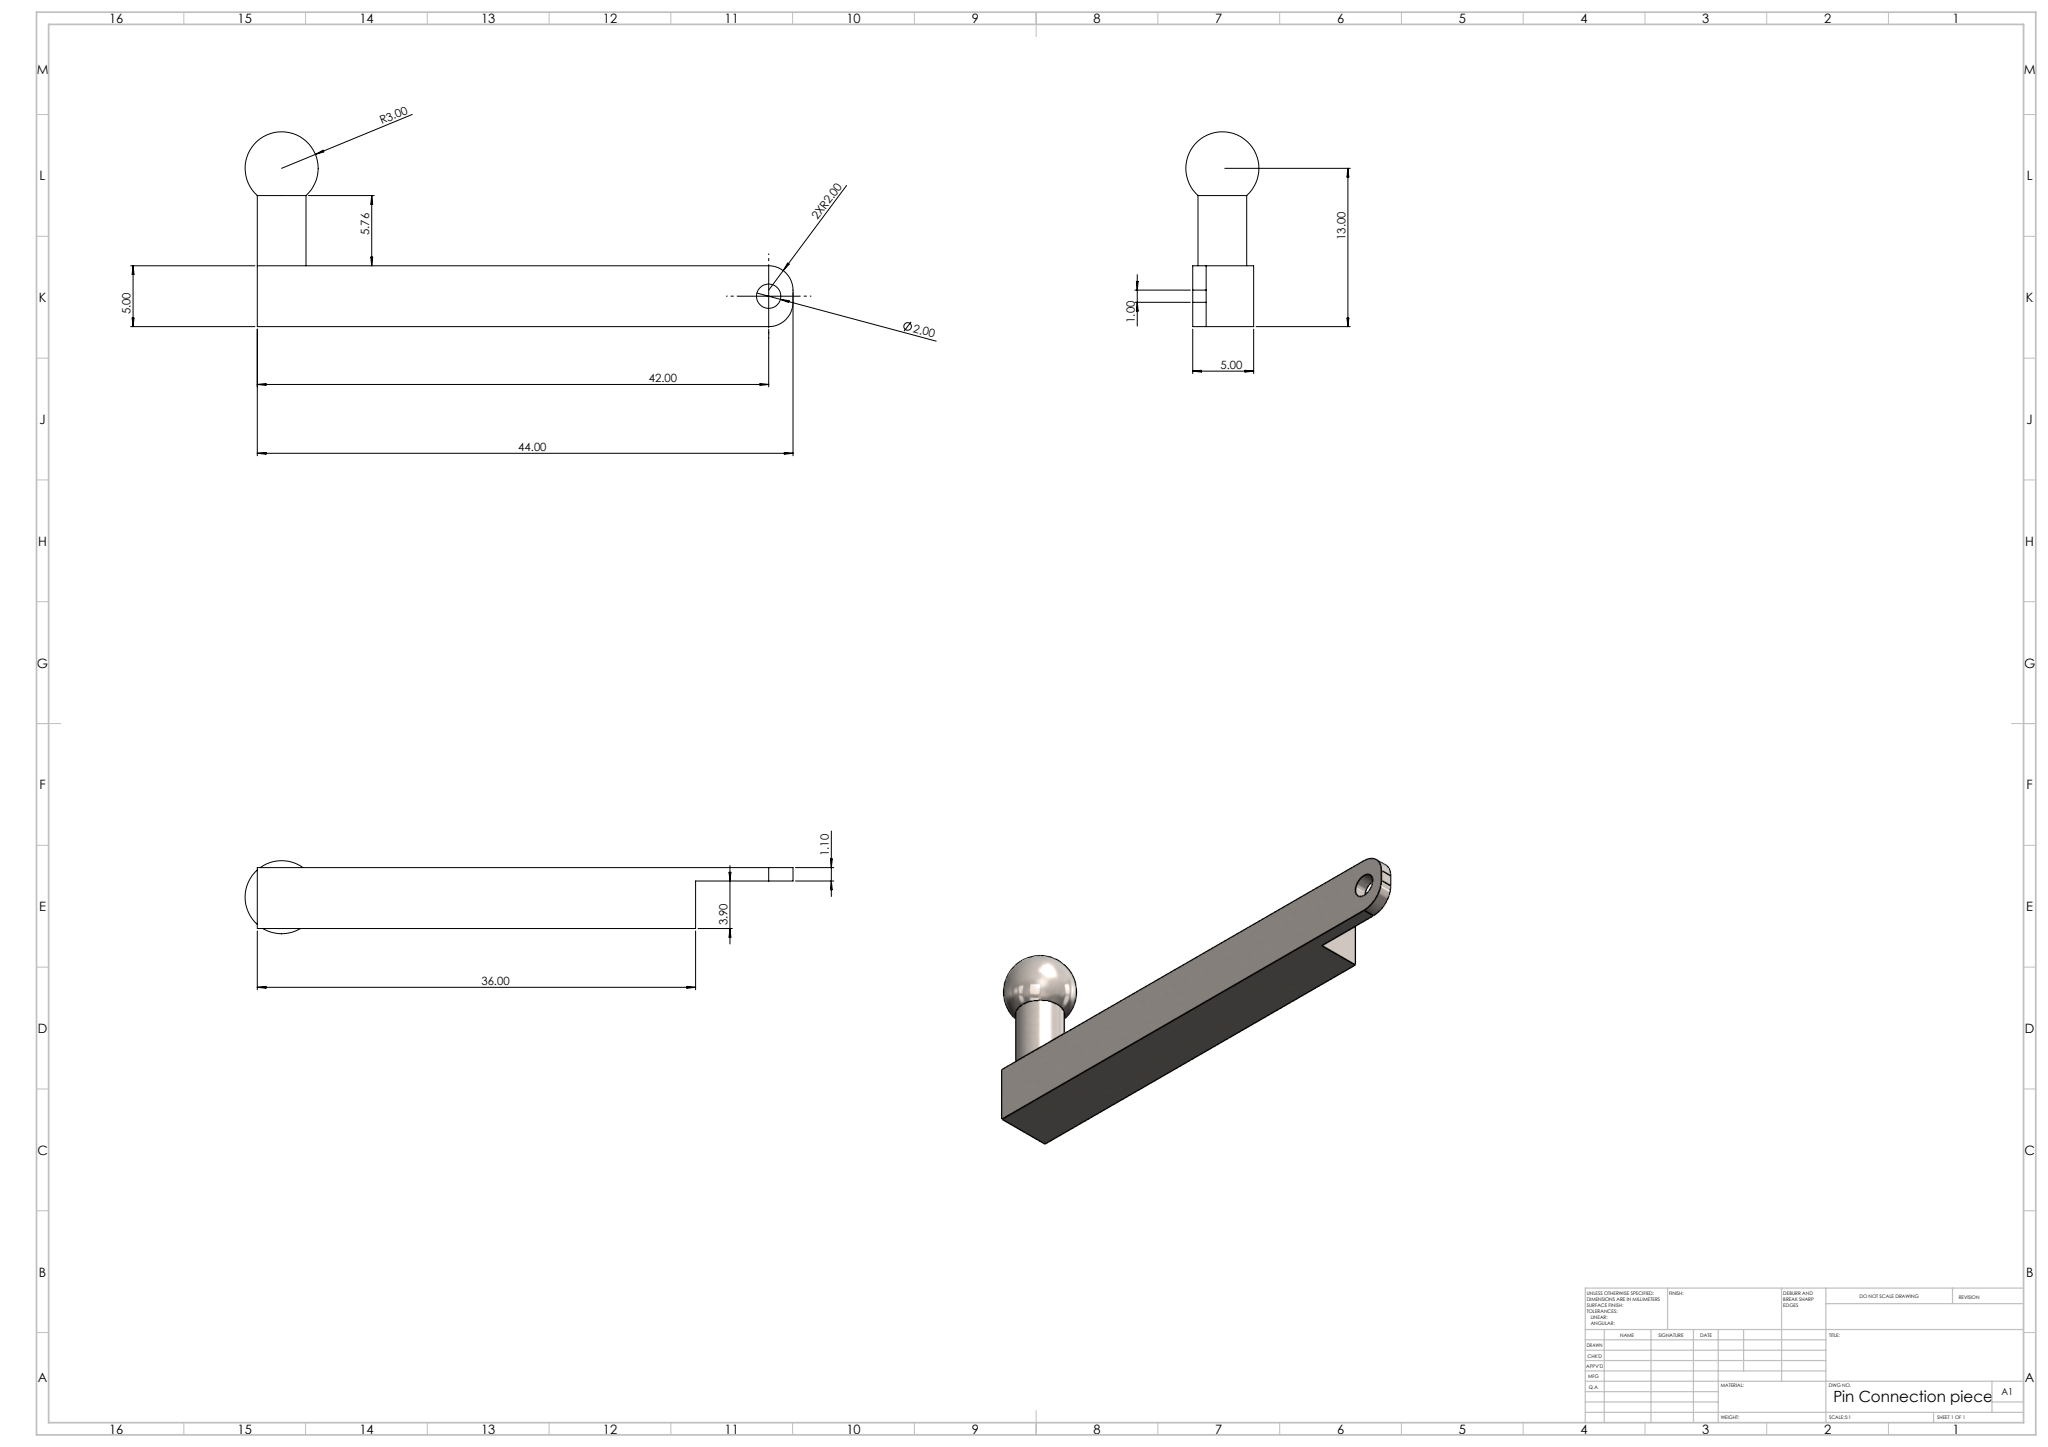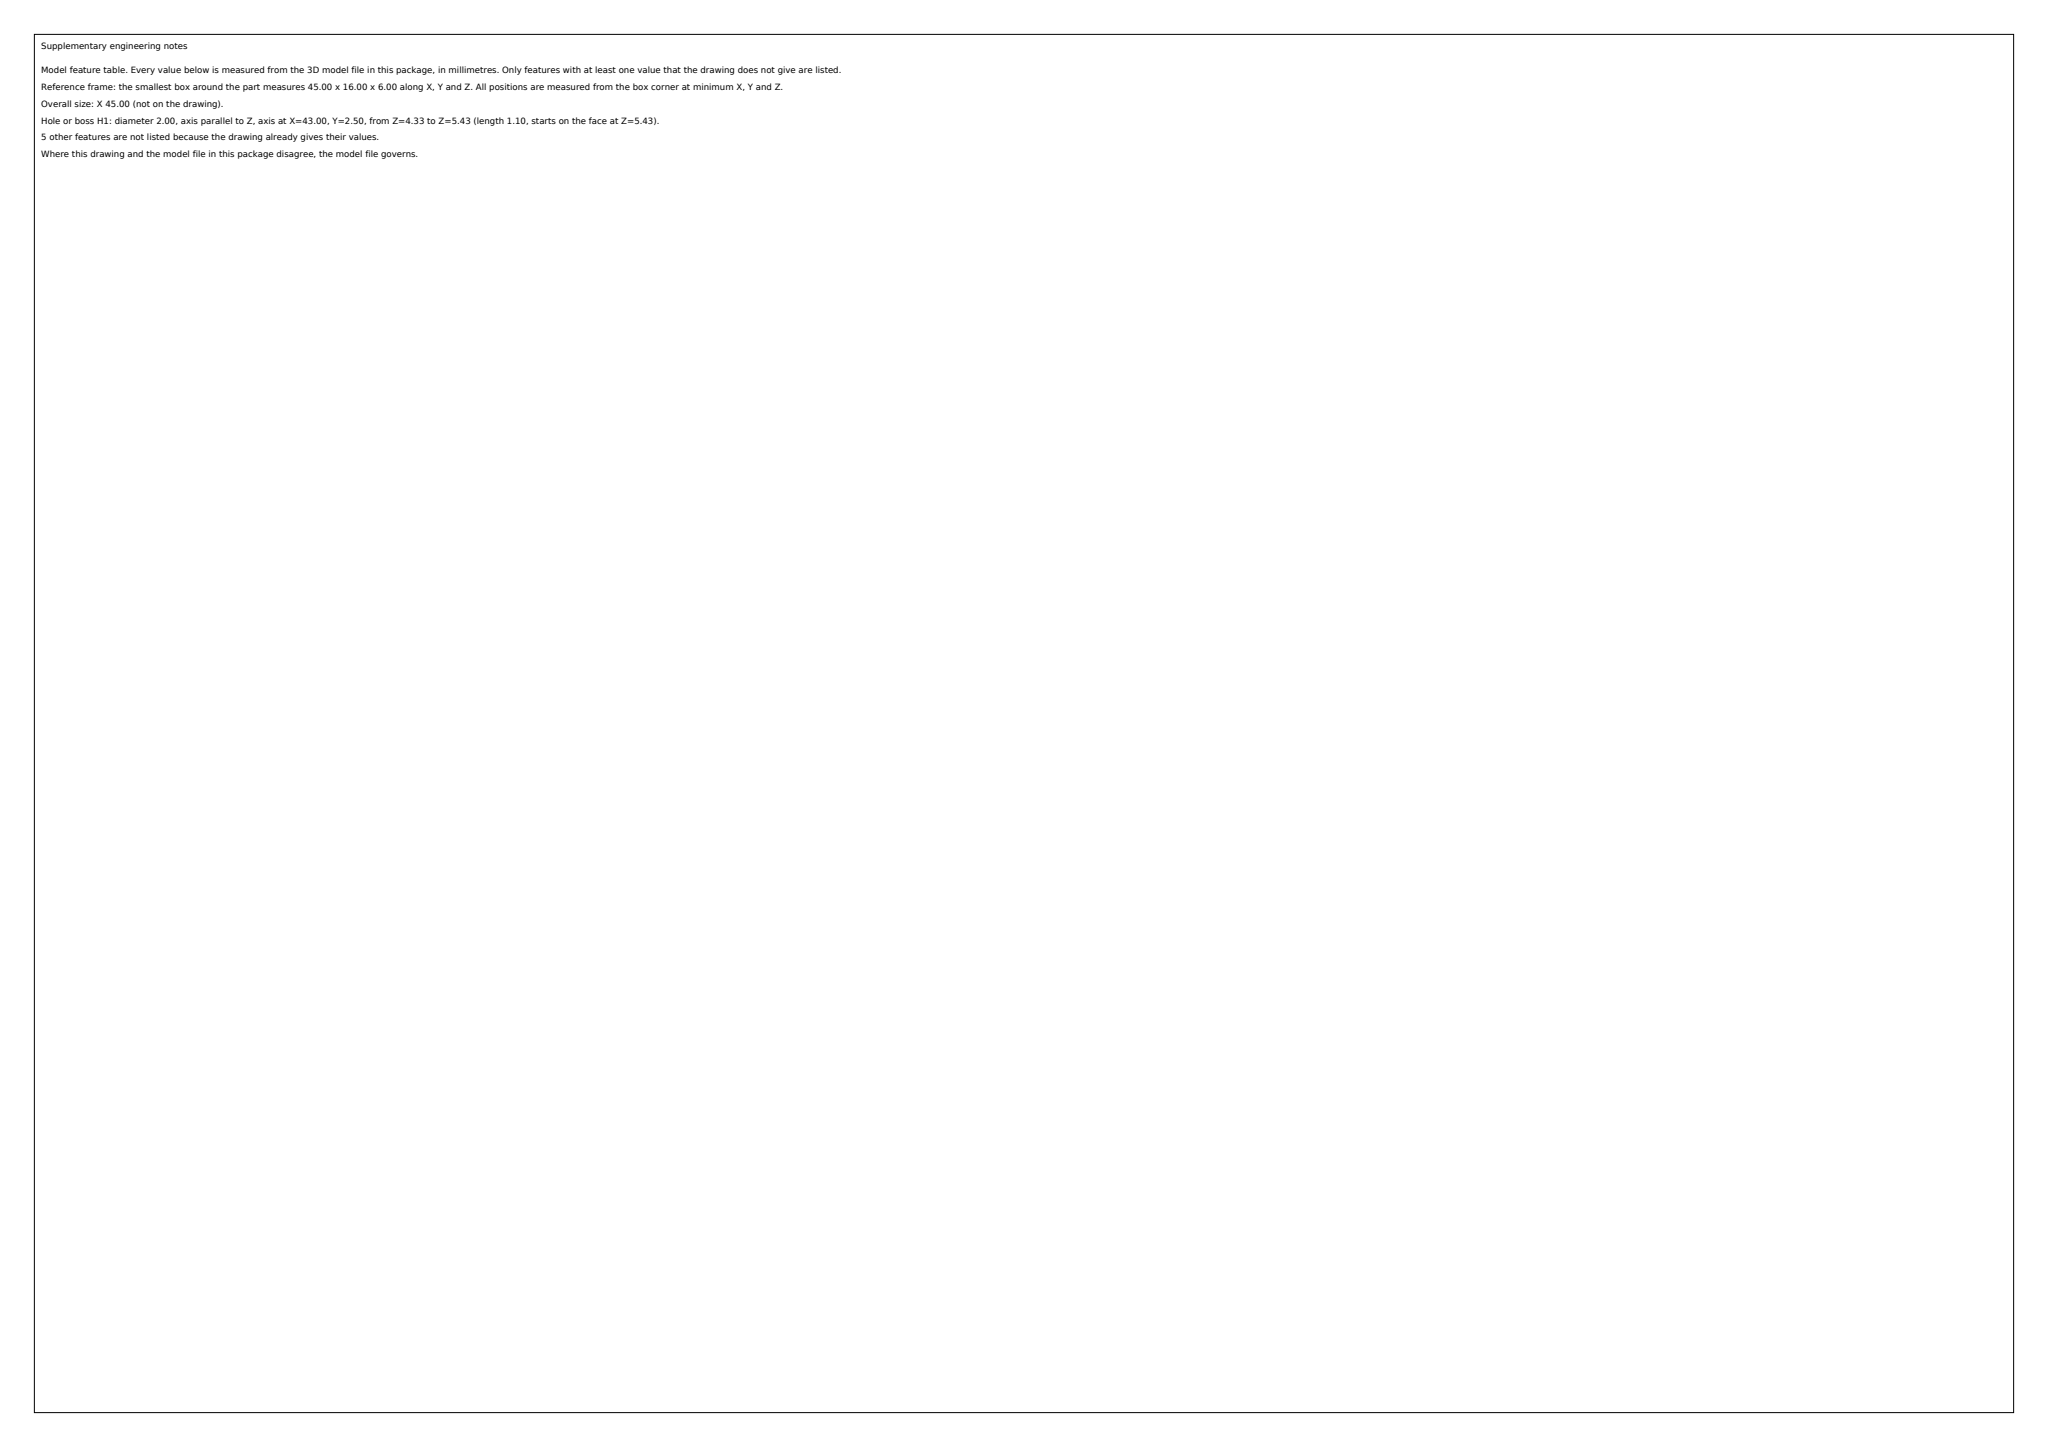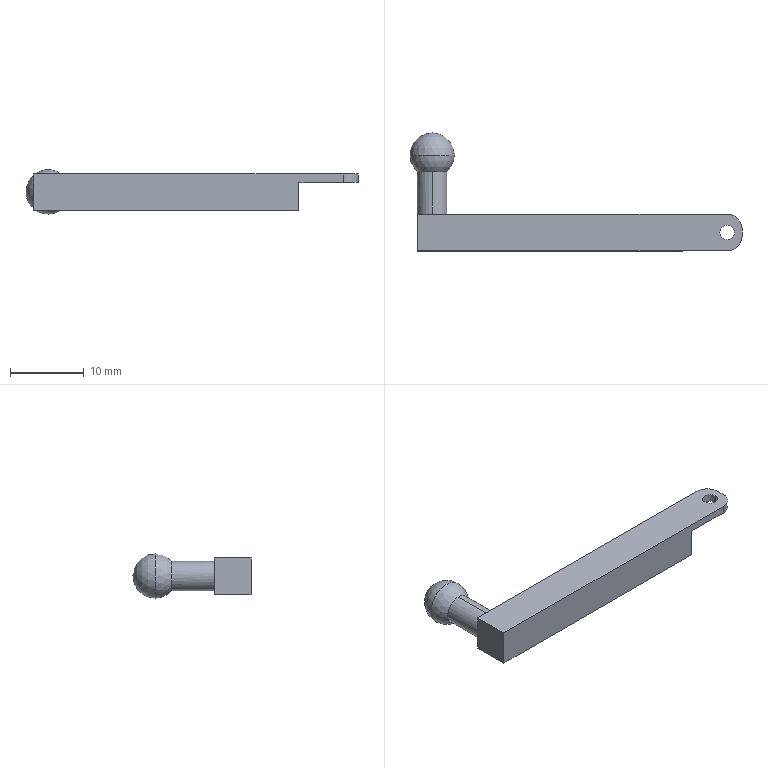Part | SolidWorks | mm | 1 solid | 16 faces | box 45 x 16 x 6 mm | volume 1119 mm3 | plane 8 | cylinder 6 | sphere 2 | commonest cylinder face diameters 4 x4 2 x2
build123d program:
from build123d import *

# Parameters (mm, degrees)
SKETCH1_W           = 36
SKETCH1_H           = 5
BOSS_EXTRUDE1_DEPTH = 5
SKETCH3_R           = 1
BOSS_EXTRUDE2_DEPTH = 1.1
SKETCH4_R           = 2
BOSS_EXTRUDE3_DEPTH = 8


with BuildPart() as part:
    # Sketch1 → Boss-Extrude1 (new body)
    with BuildSketch(Plane.XY):
        Rectangle(SKETCH1_W, SKETCH1_H)
    extrude(amount=-BOSS_EXTRUDE1_DEPTH)

    # Sketch3 → Boss-Extrude2 (add)
    with BuildSketch(Plane.XY):
        with BuildLine():
            Line((18, 2.5), (24, 2.5))
            ThreePointArc((24, 2.5), (25.414, 1.914), (26, 0.5))
            Line((26, 0.5), (26, -0.5))
            ThreePointArc((26, -0.5), (25.414, -1.914), (24, -2.5))
            Line((24, -2.5), (18, -2.5))
            Line((18, -2.5), (18, 2.5))
        make_face()
        with Locations((24, 0)):
            Circle(SKETCH3_R, mode=Mode.SUBTRACT)
    extrude(amount=-BOSS_EXTRUDE2_DEPTH)

    # Sketch4 → Boss-Extrude3 (add)
    with BuildSketch(Plane(origin=(0, 2.5, 0), x_dir=(1, 0, 0), z_dir=(0, 1, 0))):
        with Locations(Location((-16, 2.429, 0), (0, 0, 180))):
            Circle(SKETCH4_R)
    extrude(amount=BOSS_EXTRUDE3_DEPTH)

    # Sketch5 → Revolve1 (revolve)
    with BuildSketch(Plane(origin=(0, 10.5, 0), x_dir=(1, 0, 0), z_dir=(0, 1, 0))):
        with BuildLine():
            Line((-19, 2.429), (-13, 2.429))
            ThreePointArc((-13, 2.429), (-16, 5.429), (-19, 2.429))
        make_face()
    revolve(axis=Axis((-19, 10.5, -2.429), (1, 0, 0)))


solid = part.part
STEP:
#1=CARTESIAN_POINT('',(-16.,8.264,-4.429));
#2=VERTEX_POINT('',#1);
#3=CARTESIAN_POINT('',(-16.,8.264,-0.4291));
#4=VERTEX_POINT('',#3);
#5=CARTESIAN_POINT('',(-16.,8.264,-2.429));
#6=DIRECTION('',(0.,1.,0.));
#7=DIRECTION('',(0.,0.,1.));
#8=AXIS2_PLACEMENT_3D('',#5,#6,#7);
#9=CIRCLE('',#8,2.);
#10=EDGE_CURVE('',#2,#4,#9,.T.);
#11=ORIENTED_EDGE('',*,*,#10,.T.);
#12=CARTESIAN_POINT('',(-16.,8.264,-2.429));
#13=DIRECTION('',(0.,1.,0.));
#14=DIRECTION('',(0.,0.,1.));
#15=AXIS2_PLACEMENT_3D('',#12,#13,#14);
#16=CIRCLE('',#15,2.);
#17=EDGE_CURVE('',#4,#2,#16,.T.);
#18=ORIENTED_EDGE('',*,*,#17,.T.);
#19=EDGE_LOOP('',(#11,#18));
#20=FACE_BOUND('',#19,.T.);
#21=CARTESIAN_POINT('',(-13.,10.5,-2.429));
#22=VERTEX_POINT('',#21);
#23=CARTESIAN_POINT('',(-19.,10.5,-2.429));
#24=VERTEX_POINT('',#23);
#25=CARTESIAN_POINT('',(-16.,10.5,-2.429));
#26=DIRECTION('',(0.,1.,0.));
#27=DIRECTION('',(0.,0.,1.));
#28=AXIS2_PLACEMENT_3D('',#25,#26,#27);
#29=CIRCLE('',#28,3.);
#30=EDGE_CURVE('',#22,#24,#29,.T.);
#31=ORIENTED_EDGE('',*,*,#30,.F.);
#32=CARTESIAN_POINT('',(-16.,10.5,-2.429));
#33=DIRECTION('',(0.,-1.,-0.));
#34=DIRECTION('',(0.,0.,-1.));
#35=AXIS2_PLACEMENT_3D('',#32,#33,#34);
#36=CIRCLE('',#35,3.);
#37=EDGE_CURVE('',#22,#24,#36,.T.);
#38=ORIENTED_EDGE('',*,*,#37,.T.);
#39=EDGE_LOOP('',(#31,#38));
#40=FACE_OUTER_BOUND('',#39,.T.);
#41=CARTESIAN_POINT('',(-16.,10.5,-2.429));
#42=DIRECTION('',(0.,-1.,0.));
#43=DIRECTION('',(0.,0.,-1.));
#44=AXIS2_PLACEMENT_3D('',#41,#42,#43);
#45=SPHERICAL_SURFACE('',#44,3.);
#46=ADVANCED_FACE('',(#20,#40),#45,.T.);
#47=CARTESIAN_POINT('',(23.,-0.,-1.1));
#48=VERTEX_POINT('',#47);
#49=CARTESIAN_POINT('',(25.,-0.,-1.1));
#50=VERTEX_POINT('',#49);
#51=CARTESIAN_POINT('',(24.,-0.,-1.1));
#52=DIRECTION('',(0.,0.,1.));
#53=DIRECTION('',(1.,0.,0.));
#54=AXIS2_PLACEMENT_3D('',#51,#52,#53);
#55=CIRCLE('',#54,1.);
#56=EDGE_CURVE('',#48,#50,#55,.T.);
#57=ORIENTED_EDGE('',*,*,#56,.F.);
#58=CARTESIAN_POINT('',(23.,-0.,0.));
#59=VERTEX_POINT('',#58);
#60=CARTESIAN_POINT('',(23.,-0.,-1.1));
#61=DIRECTION('',(0.,0.,1.));
#62=VECTOR('',#61,1000.);
#63=LINE('',#60,#62);
#64=EDGE_CURVE('',#48,#59,#63,.T.);
#65=ORIENTED_EDGE('',*,*,#64,.T.);
#66=CARTESIAN_POINT('',(25.,-0.,0.));
#67=VERTEX_POINT('',#66);
#68=CARTESIAN_POINT('',(24.,-0.,0.));
#69=DIRECTION('',(0.,0.,1.));
#70=DIRECTION('',(1.,0.,0.));
#71=AXIS2_PLACEMENT_3D('',#68,#69,#70);
#72=CIRCLE('',#71,1.);
#73=EDGE_CURVE('',#59,#67,#72,.T.);
#74=ORIENTED_EDGE('',*,*,#73,.T.);
#75=CARTESIAN_POINT('',(25.,-0.,-1.1));
#76=DIRECTION('',(0.,0.,1.));
#77=VECTOR('',#76,1000.);
#78=LINE('',#75,#77);
#79=EDGE_CURVE('',#50,#67,#78,.T.);
#80=ORIENTED_EDGE('',*,*,#79,.F.);
#81=EDGE_LOOP('',(#57,#65,#74,#80));
#82=FACE_OUTER_BOUND('',#81,.T.);
#83=CARTESIAN_POINT('',(24.,-0.,-1.1));
#84=DIRECTION('',(0.,0.,1.));
#85=DIRECTION('',(1.,0.,0.));
#86=AXIS2_PLACEMENT_3D('',#83,#84,#85);
#87=CYLINDRICAL_SURFACE('',#86,1.);
#88=ADVANCED_FACE('',(#82),#87,.F.);
#89=ORIENTED_EDGE('',*,*,#17,.F.);
#90=CARTESIAN_POINT('',(-16.,2.5,-0.4291));
#91=VERTEX_POINT('',#90);
#92=CARTESIAN_POINT('',(-16.,10.5,-0.4291));
#93=DIRECTION('',(0.,-1.,0.));
#94=VECTOR('',#93,1000.);
#95=LINE('',#92,#94);
#96=EDGE_CURVE('',#4,#91,#95,.T.);
#97=ORIENTED_EDGE('',*,*,#96,.T.);
#98=CARTESIAN_POINT('',(-16.,2.5,-4.429));
#99=VERTEX_POINT('',#98);
#100=CARTESIAN_POINT('',(-16.,2.5,-2.429));
#101=DIRECTION('',(0.,1.,0.));
#102=DIRECTION('',(0.,0.,1.));
#103=AXIS2_PLACEMENT_3D('',#100,#101,#102);
#104=CIRCLE('',#103,2.);
#105=EDGE_CURVE('',#91,#99,#104,.T.);
#106=ORIENTED_EDGE('',*,*,#105,.T.);
#107=CARTESIAN_POINT('',(-16.,10.5,-4.429));
#108=DIRECTION('',(0.,-1.,0.));
#109=VECTOR('',#108,1000.);
#110=LINE('',#107,#109);
#111=EDGE_CURVE('',#2,#99,#110,.T.);
#112=ORIENTED_EDGE('',*,*,#111,.F.);
#113=EDGE_LOOP('',(#89,#97,#106,#112));
#114=FACE_OUTER_BOUND('',#113,.T.);
#115=CARTESIAN_POINT('',(-16.,10.5,-2.429));
#116=DIRECTION('',(0.,-1.,0.));
#117=DIRECTION('',(0.,0.,-1.));
#118=AXIS2_PLACEMENT_3D('',#115,#116,#117);
#119=CYLINDRICAL_SURFACE('',#118,2.);
#120=ADVANCED_FACE('',(#114),#119,.T.);
#121=ORIENTED_EDGE('',*,*,#96,.F.);
#122=ORIENTED_EDGE('',*,*,#10,.F.);
#123=ORIENTED_EDGE('',*,*,#111,.T.);
#124=CARTESIAN_POINT('',(-18.,2.5,-2.429));
#125=VERTEX_POINT('',#124);
#126=CARTESIAN_POINT('',(-16.,2.5,-2.429));
#127=DIRECTION('',(0.,1.,0.));
#128=DIRECTION('',(0.,0.,1.));
#129=AXIS2_PLACEMENT_3D('',#126,#127,#128);
#130=CIRCLE('',#129,2.);
#131=EDGE_CURVE('',#99,#125,#130,.T.);
#132=ORIENTED_EDGE('',*,*,#131,.T.);
#133=CARTESIAN_POINT('',(-16.,2.5,-2.429));
#134=DIRECTION('',(0.,1.,0.));
#135=DIRECTION('',(0.,0.,1.));
#136=AXIS2_PLACEMENT_3D('',#133,#134,#135);
#137=CIRCLE('',#136,2.);
#138=EDGE_CURVE('',#125,#91,#137,.T.);
#139=ORIENTED_EDGE('',*,*,#138,.T.);
#140=EDGE_LOOP('',(#121,#122,#123,#132,#139));
#141=FACE_OUTER_BOUND('',#140,.T.);
#142=CARTESIAN_POINT('',(-16.,10.5,-2.429));
#143=DIRECTION('',(0.,-1.,0.));
#144=DIRECTION('',(0.,0.,-1.));
#145=AXIS2_PLACEMENT_3D('',#142,#143,#144);
#146=CYLINDRICAL_SURFACE('',#145,2.);
#147=ADVANCED_FACE('',(#141),#146,.T.);
#148=CARTESIAN_POINT('',(18.,2.5,-5.));
#149=VERTEX_POINT('',#148);
#150=CARTESIAN_POINT('',(18.,2.5,-1.1));
#151=VERTEX_POINT('',#150);
#152=CARTESIAN_POINT('',(18.,2.5,-5.));
#153=DIRECTION('',(0.,0.,1.));
#154=VECTOR('',#153,1000.);
#155=LINE('',#152,#154);
#156=EDGE_CURVE('',#149,#151,#155,.T.);
#157=ORIENTED_EDGE('',*,*,#156,.T.);
#158=CARTESIAN_POINT('',(18.,-2.5,-1.1));
#159=VERTEX_POINT('',#158);
#160=CARTESIAN_POINT('',(18.,-2.5,-1.1));
#161=DIRECTION('',(0.,-1.,0.));
#162=VECTOR('',#161,1000.);
#163=LINE('',#160,#162);
#164=EDGE_CURVE('',#151,#159,#163,.T.);
#165=ORIENTED_EDGE('',*,*,#164,.T.);
#166=CARTESIAN_POINT('',(18.,-2.5,-5.));
#167=VERTEX_POINT('',#166);
#168=CARTESIAN_POINT('',(18.,-2.5,-5.));
#169=DIRECTION('',(0.,0.,1.));
#170=VECTOR('',#169,1000.);
#171=LINE('',#168,#170);
#172=EDGE_CURVE('',#167,#159,#171,.T.);
#173=ORIENTED_EDGE('',*,*,#172,.F.);
#174=CARTESIAN_POINT('',(18.,2.5,-5.));
#175=DIRECTION('',(0.,1.,0.));
#176=VECTOR('',#175,1000.);
#177=LINE('',#174,#176);
#178=EDGE_CURVE('',#167,#149,#177,.T.);
#179=ORIENTED_EDGE('',*,*,#178,.T.);
#180=EDGE_LOOP('',(#157,#165,#173,#179));
#181=FACE_OUTER_BOUND('',#180,.T.);
#182=CARTESIAN_POINT('',(18.,2.5,-5.));
#183=DIRECTION('',(1.,0.,0.));
#184=DIRECTION('',(0.,0.,-1.));
#185=AXIS2_PLACEMENT_3D('',#182,#183,#184);
#186=PLANE('',#185);
#187=ADVANCED_FACE('',(#181),#186,.T.);
#188=CARTESIAN_POINT('',(-18.,-2.5,0.));
#189=VERTEX_POINT('',#188);
#190=CARTESIAN_POINT('',(24.,-2.5,0.));
#191=VERTEX_POINT('',#190);
#192=CARTESIAN_POINT('',(-18.,-2.5,0.));
#193=DIRECTION('',(1.,0.,0.));
#194=VECTOR('',#193,1000.);
#195=LINE('',#192,#194);
#196=EDGE_CURVE('',#189,#191,#195,.T.);
#197=ORIENTED_EDGE('',*,*,#196,.F.);
#198=CARTESIAN_POINT('',(-18.,-2.5,-5.));
#199=VERTEX_POINT('',#198);
#200=CARTESIAN_POINT('',(-18.,-2.5,-5.));
#201=DIRECTION('',(0.,0.,1.));
#202=VECTOR('',#201,1000.);
#203=LINE('',#200,#202);
#204=EDGE_CURVE('',#199,#189,#203,.T.);
#205=ORIENTED_EDGE('',*,*,#204,.F.);
#206=CARTESIAN_POINT('',(-18.,-2.5,-5.));
#207=DIRECTION('',(1.,0.,0.));
#208=VECTOR('',#207,1000.);
#209=LINE('',#206,#208);
#210=EDGE_CURVE('',#199,#167,#209,.T.);
#211=ORIENTED_EDGE('',*,*,#210,.T.);
#212=ORIENTED_EDGE('',*,*,#172,.T.);
#213=CARTESIAN_POINT('',(24.,-2.5,-1.1));
#214=VERTEX_POINT('',#213);
#215=CARTESIAN_POINT('',(24.,-2.5,-1.1));
#216=DIRECTION('',(1.,0.,0.));
#217=VECTOR('',#216,1000.);
#218=LINE('',#215,#217);
#219=EDGE_CURVE('',#159,#214,#218,.T.);
#220=ORIENTED_EDGE('',*,*,#219,.T.);
#221=CARTESIAN_POINT('',(24.,-2.5,-1.1));
#222=DIRECTION('',(0.,0.,1.));
#223=VECTOR('',#222,1000.);
#224=LINE('',#221,#223);
#225=EDGE_CURVE('',#214,#191,#224,.T.);
#226=ORIENTED_EDGE('',*,*,#225,.T.);
#227=EDGE_LOOP('',(#197,#205,#211,#212,#220,#226));
#228=FACE_OUTER_BOUND('',#227,.T.);
#229=CARTESIAN_POINT('',(-18.,-2.5,-5.));
#230=DIRECTION('',(0.,-1.,0.));
#231=DIRECTION('',(0.,0.,-1.));
#232=AXIS2_PLACEMENT_3D('',#229,#230,#231);
#233=PLANE('',#232);
#234=ADVANCED_FACE('',(#228),#233,.T.);
#235=CARTESIAN_POINT('',(-18.,2.5,0.));
#236=VERTEX_POINT('',#235);
#237=CARTESIAN_POINT('',(-18.,2.5,0.));
#238=DIRECTION('',(0.,-1.,0.));
#239=VECTOR('',#238,1000.);
#240=LINE('',#237,#239);
#241=EDGE_CURVE('',#236,#189,#240,.T.);
#242=ORIENTED_EDGE('',*,*,#241,.F.);
#243=CARTESIAN_POINT('',(-18.,2.5,-5.));
#244=DIRECTION('',(0.,0.,1.));
#245=VECTOR('',#244,1000.);
#246=LINE('',#243,#245);
#247=EDGE_CURVE('',#125,#236,#246,.T.);
#248=ORIENTED_EDGE('',*,*,#247,.F.);
#249=CARTESIAN_POINT('',(-18.,2.5,-5.));
#250=VERTEX_POINT('',#249);
#251=CARTESIAN_POINT('',(-18.,2.5,-5.));
#252=DIRECTION('',(0.,0.,1.));
#253=VECTOR('',#252,1000.);
#254=LINE('',#251,#253);
#255=EDGE_CURVE('',#250,#125,#254,.T.);
#256=ORIENTED_EDGE('',*,*,#255,.F.);
#257=CARTESIAN_POINT('',(-18.,2.5,-5.));
#258=DIRECTION('',(0.,-1.,0.));
#259=VECTOR('',#258,1000.);
#260=LINE('',#257,#259);
#261=EDGE_CURVE('',#250,#199,#260,.T.);
#262=ORIENTED_EDGE('',*,*,#261,.T.);
#263=ORIENTED_EDGE('',*,*,#204,.T.);
#264=EDGE_LOOP('',(#242,#248,#256,#262,#263));
#265=FACE_OUTER_BOUND('',#264,.T.);
#266=CARTESIAN_POINT('',(-18.,2.5,-5.));
#267=DIRECTION('',(-1.,0.,0.));
#268=DIRECTION('',(0.,0.,1.));
#269=AXIS2_PLACEMENT_3D('',#266,#267,#268);
#270=PLANE('',#269);
#271=ADVANCED_FACE('',(#265),#270,.T.);
#272=ORIENTED_EDGE('',*,*,#255,.T.);
#273=ORIENTED_EDGE('',*,*,#131,.F.);
#274=ORIENTED_EDGE('',*,*,#105,.F.);
#275=ORIENTED_EDGE('',*,*,#138,.F.);
#276=ORIENTED_EDGE('',*,*,#247,.T.);
#277=CARTESIAN_POINT('',(24.,2.5,0.));
#278=VERTEX_POINT('',#277);
#279=CARTESIAN_POINT('',(-18.,2.5,0.));
#280=DIRECTION('',(-1.,0.,0.));
#281=VECTOR('',#280,1000.);
#282=LINE('',#279,#281);
#283=EDGE_CURVE('',#278,#236,#282,.T.);
#284=ORIENTED_EDGE('',*,*,#283,.F.);
#285=CARTESIAN_POINT('',(24.,2.5,-1.1));
#286=VERTEX_POINT('',#285);
#287=CARTESIAN_POINT('',(24.,2.5,-1.1));
#288=DIRECTION('',(0.,0.,1.));
#289=VECTOR('',#288,1000.);
#290=LINE('',#287,#289);
#291=EDGE_CURVE('',#286,#278,#290,.T.);
#292=ORIENTED_EDGE('',*,*,#291,.F.);
#293=CARTESIAN_POINT('',(18.,2.5,-1.1));
#294=DIRECTION('',(-1.,0.,0.));
#295=VECTOR('',#294,1000.);
#296=LINE('',#293,#295);
#297=EDGE_CURVE('',#286,#151,#296,.T.);
#298=ORIENTED_EDGE('',*,*,#297,.T.);
#299=ORIENTED_EDGE('',*,*,#156,.F.);
#300=CARTESIAN_POINT('',(-18.,2.5,-5.));
#301=DIRECTION('',(-1.,0.,0.));
#302=VECTOR('',#301,1000.);
#303=LINE('',#300,#302);
#304=EDGE_CURVE('',#149,#250,#303,.T.);
#305=ORIENTED_EDGE('',*,*,#304,.T.);
#306=EDGE_LOOP('',(#272,#273,#274,#275,#276,#284,#292,#298,#299,#305));
#307=FACE_OUTER_BOUND('',#306,.T.);
#308=CARTESIAN_POINT('',(-18.,2.5,-5.));
#309=DIRECTION('',(0.,1.,0.));
#310=DIRECTION('',(0.,0.,1.));
#311=AXIS2_PLACEMENT_3D('',#308,#309,#310);
#312=PLANE('',#311);
#313=ADVANCED_FACE('',(#307),#312,.T.);
#314=ORIENTED_EDGE('',*,*,#178,.F.);
#315=ORIENTED_EDGE('',*,*,#210,.F.);
#316=ORIENTED_EDGE('',*,*,#261,.F.);
#317=ORIENTED_EDGE('',*,*,#304,.F.);
#318=EDGE_LOOP('',(#314,#315,#316,#317));
#319=FACE_OUTER_BOUND('',#318,.T.);
#320=CARTESIAN_POINT('',(0.,0.,-5.));
#321=DIRECTION('',(0.,0.,1.));
#322=DIRECTION('',(1.,0.,0.));
#323=AXIS2_PLACEMENT_3D('',#320,#321,#322);
#324=PLANE('',#323);
#325=ADVANCED_FACE('',(#319),#324,.F.);
#326=ORIENTED_EDGE('',*,*,#196,.T.);
#327=CARTESIAN_POINT('',(26.,-0.5,0.));
#328=VERTEX_POINT('',#327);
#329=CARTESIAN_POINT('',(24.,-0.5,0.));
#330=DIRECTION('',(0.,0.,1.));
#331=DIRECTION('',(1.,0.,0.));
#332=AXIS2_PLACEMENT_3D('',#329,#330,#331);
#333=CIRCLE('',#332,2.);
#334=EDGE_CURVE('',#191,#328,#333,.T.);
#335=ORIENTED_EDGE('',*,*,#334,.T.);
#336=CARTESIAN_POINT('',(26.,0.5,0.));
#337=VERTEX_POINT('',#336);
#338=CARTESIAN_POINT('',(26.,0.5,0.));
#339=DIRECTION('',(0.,1.,0.));
#340=VECTOR('',#339,1000.);
#341=LINE('',#338,#340);
#342=EDGE_CURVE('',#328,#337,#341,.T.);
#343=ORIENTED_EDGE('',*,*,#342,.T.);
#344=CARTESIAN_POINT('',(24.,0.5,0.));
#345=DIRECTION('',(0.,0.,1.));
#346=DIRECTION('',(1.,0.,0.));
#347=AXIS2_PLACEMENT_3D('',#344,#345,#346);
#348=CIRCLE('',#347,2.);
#349=EDGE_CURVE('',#337,#278,#348,.T.);
#350=ORIENTED_EDGE('',*,*,#349,.T.);
#351=ORIENTED_EDGE('',*,*,#283,.T.);
#352=ORIENTED_EDGE('',*,*,#241,.T.);
#353=EDGE_LOOP('',(#326,#335,#343,#350,#351,#352));
#354=FACE_OUTER_BOUND('',#353,.T.);
#355=CARTESIAN_POINT('',(24.,-0.,0.));
#356=DIRECTION('',(0.,0.,1.));
#357=DIRECTION('',(1.,0.,0.));
#358=AXIS2_PLACEMENT_3D('',#355,#356,#357);
#359=CIRCLE('',#358,1.);
#360=EDGE_CURVE('',#67,#59,#359,.T.);
#361=ORIENTED_EDGE('',*,*,#360,.F.);
#362=ORIENTED_EDGE('',*,*,#73,.F.);
#363=EDGE_LOOP('',(#361,#362));
#364=FACE_BOUND('',#363,.T.);
#365=CARTESIAN_POINT('',(0.,0.,0.));
#366=DIRECTION('',(0.,0.,1.));
#367=DIRECTION('',(1.,0.,0.));
#368=AXIS2_PLACEMENT_3D('',#365,#366,#367);
#369=PLANE('',#368);
#370=ADVANCED_FACE('',(#354,#364),#369,.T.);
#371=ORIENTED_EDGE('',*,*,#349,.F.);
#372=CARTESIAN_POINT('',(26.,0.5,-1.1));
#373=VERTEX_POINT('',#372);
#374=CARTESIAN_POINT('',(26.,0.5,-1.1));
#375=DIRECTION('',(0.,0.,1.));
#376=VECTOR('',#375,1000.);
#377=LINE('',#374,#376);
#378=EDGE_CURVE('',#373,#337,#377,.T.);
#379=ORIENTED_EDGE('',*,*,#378,.F.);
#380=CARTESIAN_POINT('',(24.,0.5,-1.1));
#381=DIRECTION('',(0.,0.,1.));
#382=DIRECTION('',(1.,0.,0.));
#383=AXIS2_PLACEMENT_3D('',#380,#381,#382);
#384=CIRCLE('',#383,2.);
#385=EDGE_CURVE('',#373,#286,#384,.T.);
#386=ORIENTED_EDGE('',*,*,#385,.T.);
#387=ORIENTED_EDGE('',*,*,#291,.T.);
#388=EDGE_LOOP('',(#371,#379,#386,#387));
#389=FACE_OUTER_BOUND('',#388,.T.);
#390=CARTESIAN_POINT('',(24.,0.5,-1.1));
#391=DIRECTION('',(0.,0.,1.));
#392=DIRECTION('',(1.,0.,0.));
#393=AXIS2_PLACEMENT_3D('',#390,#391,#392);
#394=CYLINDRICAL_SURFACE('',#393,2.);
#395=ADVANCED_FACE('',(#389),#394,.T.);
#396=ORIENTED_EDGE('',*,*,#342,.F.);
#397=CARTESIAN_POINT('',(26.,-0.5,-1.1));
#398=VERTEX_POINT('',#397);
#399=CARTESIAN_POINT('',(26.,-0.5,-1.1));
#400=DIRECTION('',(0.,0.,1.));
#401=VECTOR('',#400,1000.);
#402=LINE('',#399,#401);
#403=EDGE_CURVE('',#398,#328,#402,.T.);
#404=ORIENTED_EDGE('',*,*,#403,.F.);
#405=CARTESIAN_POINT('',(26.,0.5,-1.1));
#406=DIRECTION('',(0.,1.,0.));
#407=VECTOR('',#406,1000.);
#408=LINE('',#405,#407);
#409=EDGE_CURVE('',#398,#373,#408,.T.);
#410=ORIENTED_EDGE('',*,*,#409,.T.);
#411=ORIENTED_EDGE('',*,*,#378,.T.);
#412=EDGE_LOOP('',(#396,#404,#410,#411));
#413=FACE_OUTER_BOUND('',#412,.T.);
#414=CARTESIAN_POINT('',(26.,0.5,-1.1));
#415=DIRECTION('',(1.,0.,0.));
#416=DIRECTION('',(0.,0.,-1.));
#417=AXIS2_PLACEMENT_3D('',#414,#415,#416);
#418=PLANE('',#417);
#419=ADVANCED_FACE('',(#413),#418,.T.);
#420=ORIENTED_EDGE('',*,*,#334,.F.);
#421=ORIENTED_EDGE('',*,*,#225,.F.);
#422=CARTESIAN_POINT('',(24.,-0.5,-1.1));
#423=DIRECTION('',(0.,0.,1.));
#424=DIRECTION('',(1.,0.,0.));
#425=AXIS2_PLACEMENT_3D('',#422,#423,#424);
#426=CIRCLE('',#425,2.);
#427=EDGE_CURVE('',#214,#398,#426,.T.);
#428=ORIENTED_EDGE('',*,*,#427,.T.);
#429=ORIENTED_EDGE('',*,*,#403,.T.);
#430=EDGE_LOOP('',(#420,#421,#428,#429));
#431=FACE_OUTER_BOUND('',#430,.T.);
#432=CARTESIAN_POINT('',(24.,-0.5,-1.1));
#433=DIRECTION('',(0.,0.,1.));
#434=DIRECTION('',(1.,0.,0.));
#435=AXIS2_PLACEMENT_3D('',#432,#433,#434);
#436=CYLINDRICAL_SURFACE('',#435,2.);
#437=ADVANCED_FACE('',(#431),#436,.T.);
#438=CARTESIAN_POINT('',(24.,-0.,-1.1));
#439=DIRECTION('',(0.,0.,1.));
#440=DIRECTION('',(1.,0.,0.));
#441=AXIS2_PLACEMENT_3D('',#438,#439,#440);
#442=CIRCLE('',#441,1.);
#443=EDGE_CURVE('',#50,#48,#442,.T.);
#444=ORIENTED_EDGE('',*,*,#443,.T.);
#445=ORIENTED_EDGE('',*,*,#56,.T.);
#446=EDGE_LOOP('',(#444,#445));
#447=FACE_BOUND('',#446,.T.);
#448=ORIENTED_EDGE('',*,*,#164,.F.);
#449=ORIENTED_EDGE('',*,*,#297,.F.);
#450=ORIENTED_EDGE('',*,*,#385,.F.);
#451=ORIENTED_EDGE('',*,*,#409,.F.);
#452=ORIENTED_EDGE('',*,*,#427,.F.);
#453=ORIENTED_EDGE('',*,*,#219,.F.);
#454=EDGE_LOOP('',(#448,#449,#450,#451,#452,#453));
#455=FACE_OUTER_BOUND('',#454,.T.);
#456=CARTESIAN_POINT('',(24.,0.5,-1.1));
#457=DIRECTION('',(0.,0.,1.));
#458=DIRECTION('',(1.,0.,0.));
#459=AXIS2_PLACEMENT_3D('',#456,#457,#458);
#460=PLANE('',#459);
#461=ADVANCED_FACE('',(#447,#455),#460,.F.);
#462=ORIENTED_EDGE('',*,*,#64,.F.);
#463=ORIENTED_EDGE('',*,*,#443,.F.);
#464=ORIENTED_EDGE('',*,*,#79,.T.);
#465=ORIENTED_EDGE('',*,*,#360,.T.);
#466=EDGE_LOOP('',(#462,#463,#464,#465));
#467=FACE_OUTER_BOUND('',#466,.T.);
#468=CARTESIAN_POINT('',(24.,-0.,-1.1));
#469=DIRECTION('',(0.,0.,1.));
#470=DIRECTION('',(1.,0.,0.));
#471=AXIS2_PLACEMENT_3D('',#468,#469,#470);
#472=CYLINDRICAL_SURFACE('',#471,1.);
#473=ADVANCED_FACE('',(#467),#472,.F.);
#474=ORIENTED_EDGE('',*,*,#37,.F.);
#475=ORIENTED_EDGE('',*,*,#30,.T.);
#476=EDGE_LOOP('',(#474,#475));
#477=FACE_OUTER_BOUND('',#476,.T.);
#478=CARTESIAN_POINT('',(-16.,10.5,-2.429));
#479=DIRECTION('',(0.,-1.,0.));
#480=DIRECTION('',(0.,0.,-1.));
#481=AXIS2_PLACEMENT_3D('',#478,#479,#480);
#482=SPHERICAL_SURFACE('',#481,3.);
#483=ADVANCED_FACE('',(#477),#482,.T.);
#484=CLOSED_SHELL('',(#46,#88,#120,#147,#187,#234,#271,#313,#325,#370,#395,#419,#437,#461,#473,#483));
#485=MANIFOLD_SOLID_BREP('',#484);
#486=CARTESIAN_POINT('',(0.,0.,0.));
#487=DIRECTION('',(0.,0.,1.));
#488=DIRECTION('',(1.,0.,0.));
#489=AXIS2_PLACEMENT_3D('',#486,#487,#488);
#490=(LENGTH_UNIT()NAMED_UNIT(*)SI_UNIT(.MILLI.,.METRE.));
#491=UNCERTAINTY_MEASURE_WITH_UNIT(LENGTH_MEASURE(0.00001),#490,'','');
#492=(NAMED_UNIT(*)PLANE_ANGLE_UNIT()SI_UNIT($,.RADIAN.));
#493=(NAMED_UNIT(*)SI_UNIT($,.STERADIAN.)SOLID_ANGLE_UNIT());
#494=(GEOMETRIC_REPRESENTATION_CONTEXT(3)GLOBAL_UNCERTAINTY_ASSIGNED_CONTEXT((#491))GLOBAL_UNIT_ASSIGNED_CONTEXT((#490,#492,#493))REPRESENTATION_CONTEXT('',''));
#495=ADVANCED_BREP_SHAPE_REPRESENTATION('',(#485,#489),#494);